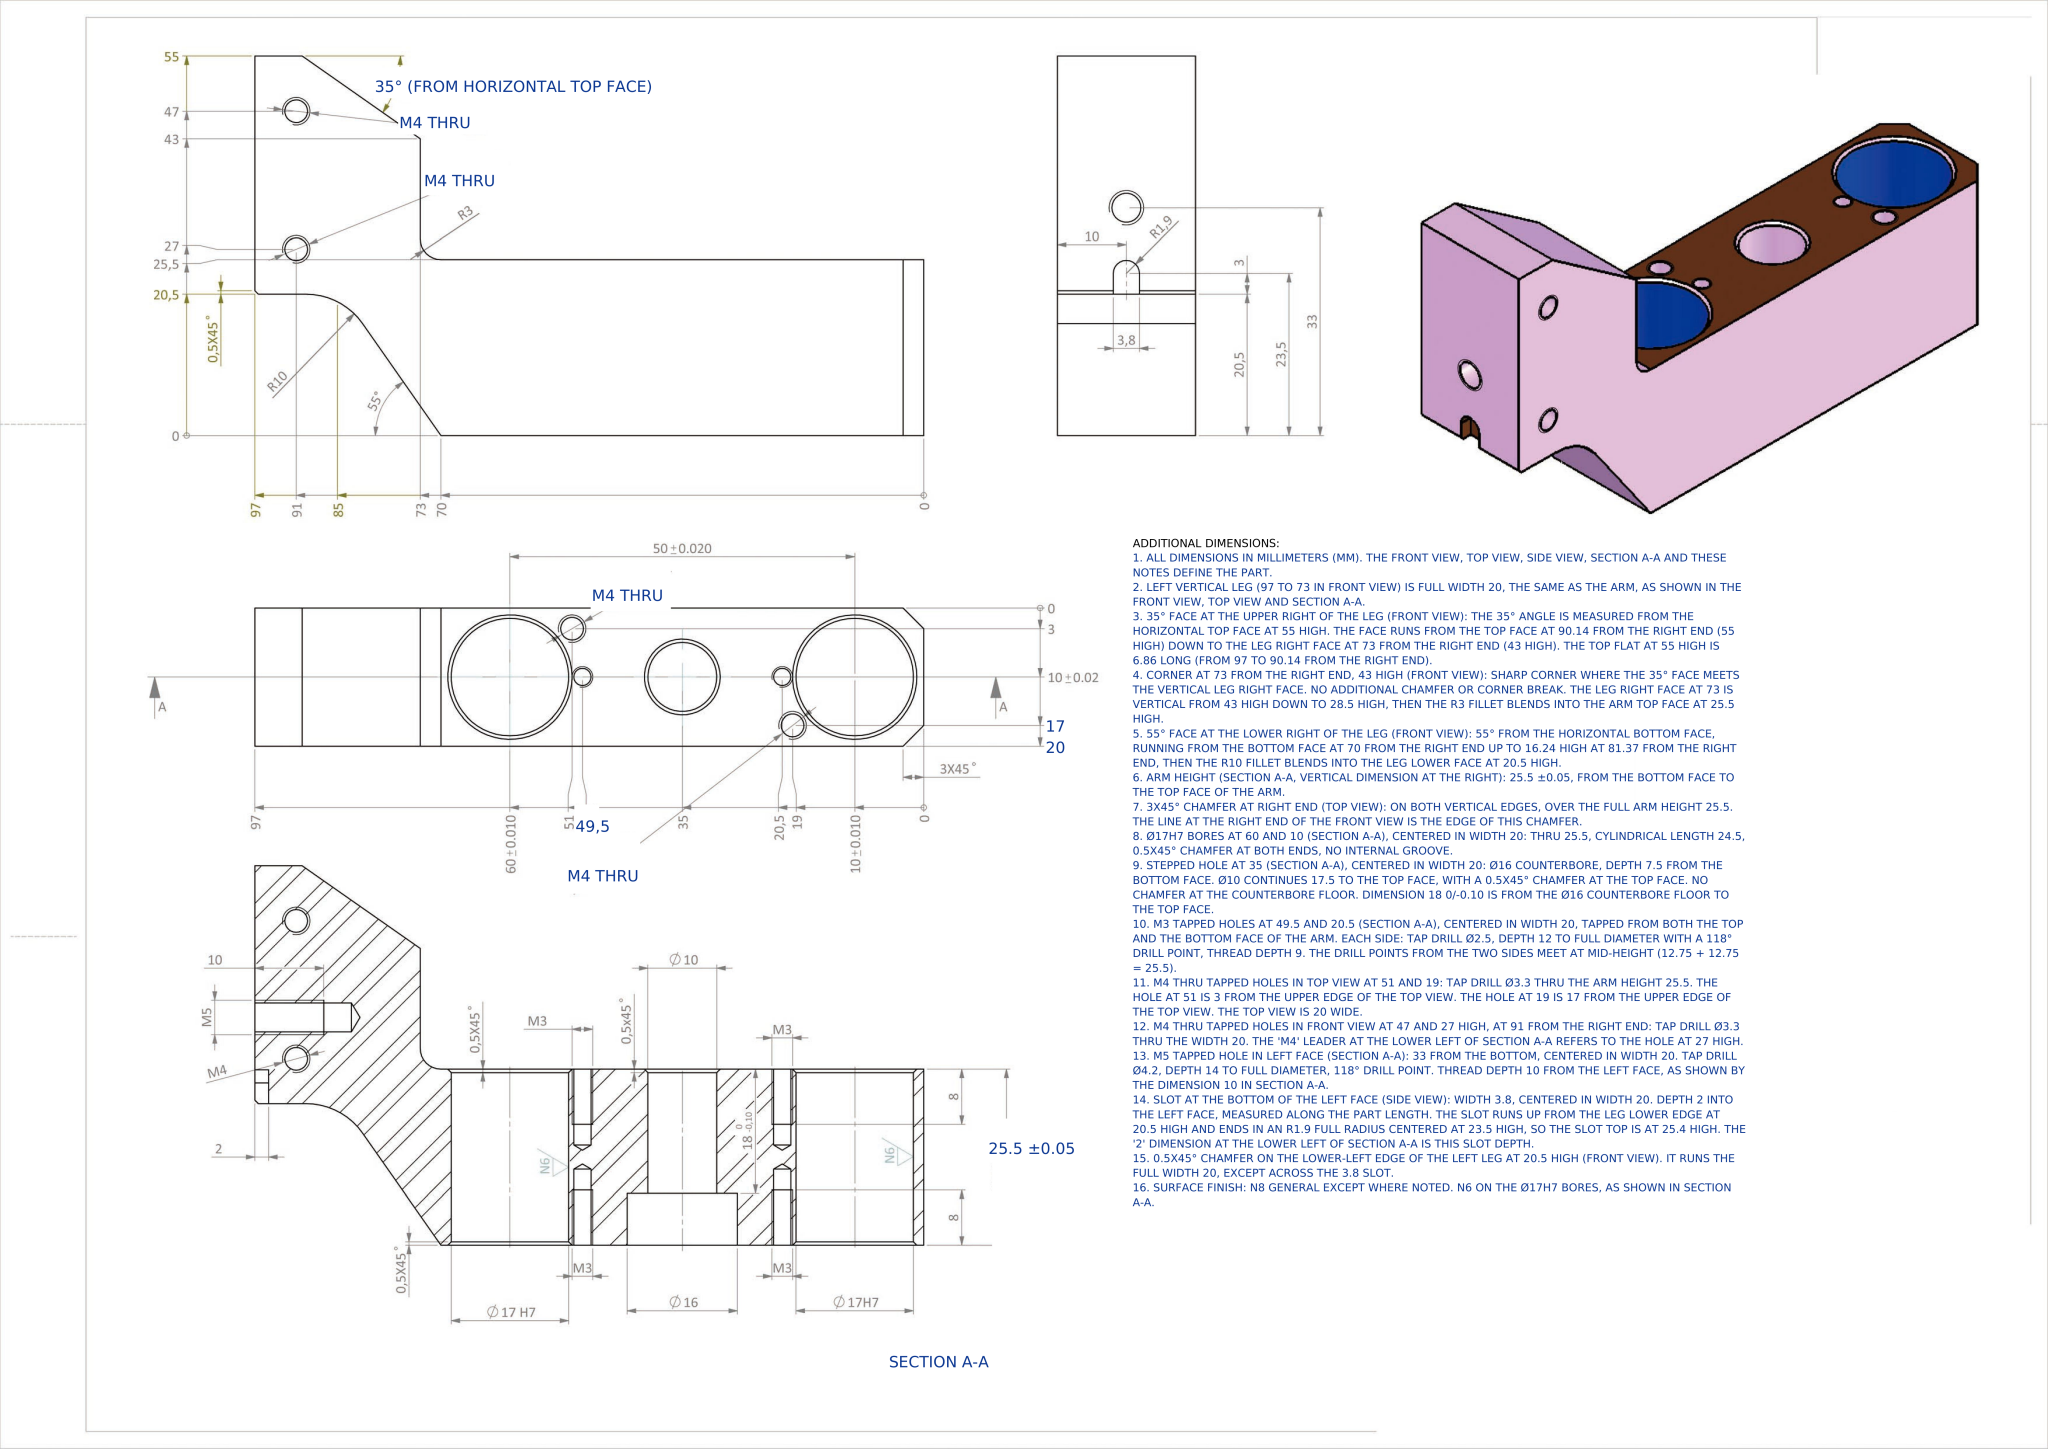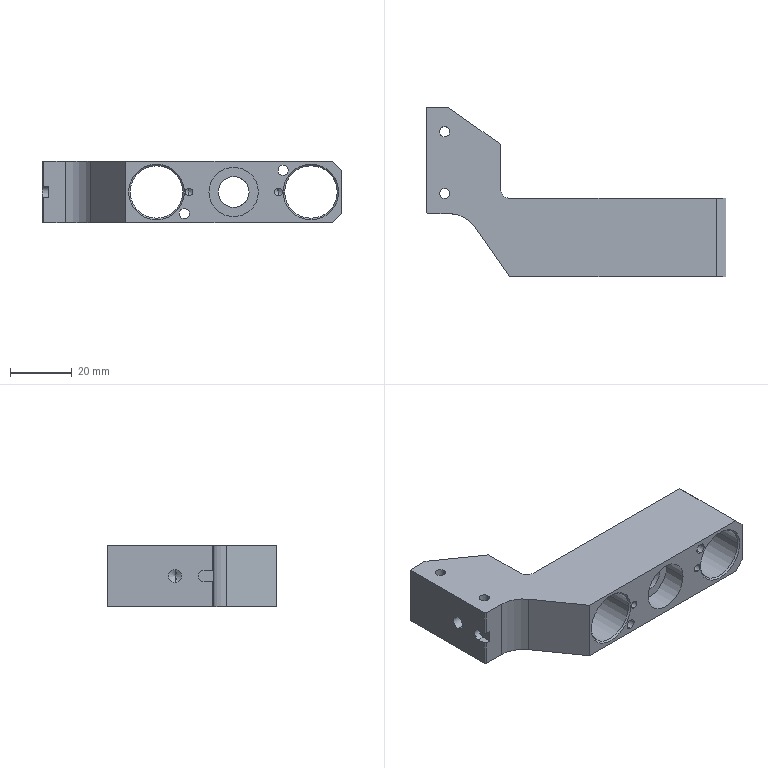Part | NX | mm | 1 solid | 68 faces | box 97 x 55 x 20 mm | volume 37572 mm3 | cylinder 29 | cone 20 | plane 19 | commonest cylinder face diameters 3.3 x8 2.5 x8 17 x4 4.2 x2 16 x2 10 x2 3.8 x1 6 x1